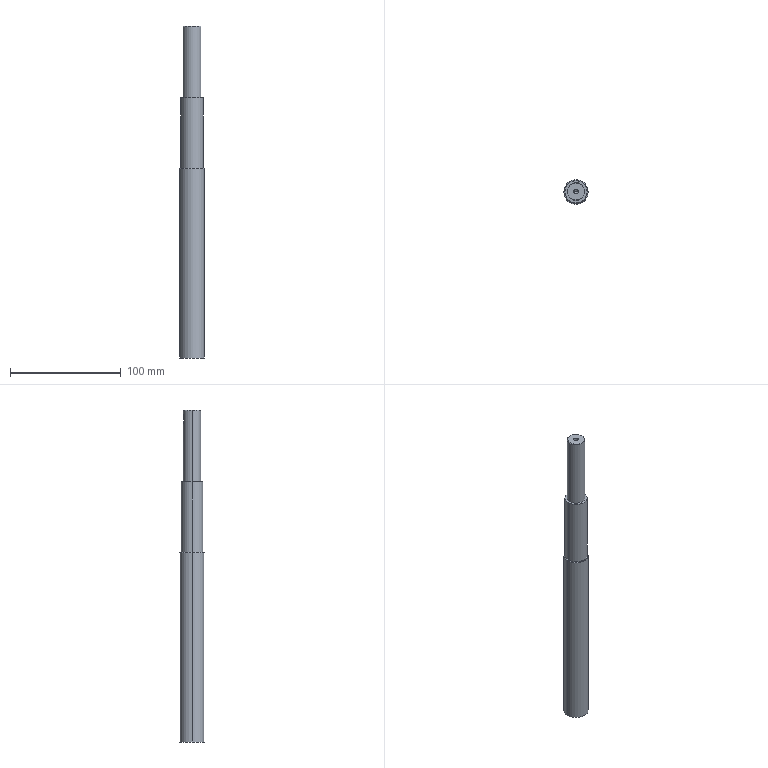Component | SolidWorks | UpperSideBeltRisingScrewXG-XG1-1 | 1 solid | 23 faces | box 22 x 22 x 300 mm | volume 97876 mm3 | cylinder 10 | plane 7 | cone 6 | commonest cylinder face diameters 4.2 x2 16 x2 20 x2 22 x2 5 x2
STEP:
#1=CARTESIAN_POINT('',(-13.812,18.504,15.591));
#2=VERTEX_POINT('',#1);
#3=CARTESIAN_POINT('',(-13.646,18.504,15.591));
#4=VERTEX_POINT('',#3);
#5=CARTESIAN_POINT('',(-13.729,18.504,15.591));
#6=DIRECTION('',(0.,-0.,1.));
#7=DIRECTION('',(1.,0.,0.));
#8=AXIS2_PLACEMENT_3D('',#5,#6,#7);
#9=CIRCLE('',#8,0.08268);
#10=EDGE_CURVE('',#2,#4,#9,.T.);
#11=ORIENTED_EDGE('',*,*,#10,.F.);
#12=CARTESIAN_POINT('',(-13.812,18.504,16.08));
#13=VERTEX_POINT('',#12);
#14=CARTESIAN_POINT('',(-13.812,18.504,16.08));
#15=DIRECTION('',(0.,-0.,1.));
#16=VECTOR('',#15,39.37);
#17=LINE('',#14,#16);
#18=EDGE_CURVE('',#2,#13,#17,.T.);
#19=ORIENTED_EDGE('',*,*,#18,.T.);
#20=CARTESIAN_POINT('',(-13.646,18.504,16.08));
#21=VERTEX_POINT('',#20);
#22=CARTESIAN_POINT('',(-13.729,18.504,16.08));
#23=DIRECTION('',(0.,-0.,1.));
#24=DIRECTION('',(1.,0.,0.));
#25=AXIS2_PLACEMENT_3D('',#22,#23,#24);
#26=CIRCLE('',#25,0.08268);
#27=EDGE_CURVE('',#13,#21,#26,.T.);
#28=ORIENTED_EDGE('',*,*,#27,.T.);
#29=CARTESIAN_POINT('',(-13.646,18.504,16.08));
#30=DIRECTION('',(0.,-0.,1.));
#31=VECTOR('',#30,39.37);
#32=LINE('',#29,#31);
#33=EDGE_CURVE('',#4,#21,#32,.T.);
#34=ORIENTED_EDGE('',*,*,#33,.F.);
#35=EDGE_LOOP('',(#11,#19,#28,#34));
#36=FACE_OUTER_BOUND('',#35,.T.);
#37=CARTESIAN_POINT('',(-13.729,18.504,16.08));
#38=DIRECTION('',(0.,-0.,1.));
#39=DIRECTION('',(1.,0.,0.));
#40=AXIS2_PLACEMENT_3D('',#37,#38,#39);
#41=CYLINDRICAL_SURFACE('',#40,0.08268);
#42=ADVANCED_FACE('',(#36),#41,.F.);
#43=CARTESIAN_POINT('',(-13.729,18.504,15.542));
#44=VERTEX_POINT('',#43);
#45=CARTESIAN_POINT('',(-13.646,18.504,15.591));
#46=DIRECTION('',(0.8572,-0.,0.515));
#47=VECTOR('',#46,39.37);
#48=LINE('',#45,#47);
#49=EDGE_CURVE('',#44,#4,#48,.T.);
#50=ORIENTED_EDGE('',*,*,#49,.F.);
#51=CARTESIAN_POINT('',(-13.812,18.504,15.591));
#52=DIRECTION('',(-0.8572,-0.,0.515));
#53=VECTOR('',#52,39.37);
#54=LINE('',#51,#53);
#55=EDGE_CURVE('',#44,#2,#54,.T.);
#56=ORIENTED_EDGE('',*,*,#55,.T.);
#57=ORIENTED_EDGE('',*,*,#10,.T.);
#58=EDGE_LOOP('',(#50,#56,#57));
#59=FACE_OUTER_BOUND('',#58,.T.);
#60=CARTESIAN_POINT('',(-13.729,18.504,15.591));
#61=DIRECTION('',(0.,-0.,1.));
#62=DIRECTION('',(1.,0.,0.));
#63=AXIS2_PLACEMENT_3D('',#60,#61,#62);
#64=CONICAL_SURFACE('',#63,0.08268,1.03);
#65=ADVANCED_FACE('',(#59),#64,.F.);
#66=CARTESIAN_POINT('',(-13.828,18.803,15.883));
#67=VERTEX_POINT('',#66);
#68=CARTESIAN_POINT('',(-13.828,18.803,15.646));
#69=VERTEX_POINT('',#68);
#70=CARTESIAN_POINT('',(-13.828,18.803,16.97));
#71=DIRECTION('',(-0.,0.,-1.));
#72=VECTOR('',#71,39.37);
#73=LINE('',#70,#72);
#74=EDGE_CURVE('',#67,#69,#73,.T.);
#75=ORIENTED_EDGE('',*,*,#74,.T.);
#76=CARTESIAN_POINT('',(-13.631,18.803,15.646));
#77=VERTEX_POINT('',#76);
#78=CARTESIAN_POINT('',(-13.828,18.803,15.646));
#79=CARTESIAN_POINT('',(-13.828,18.803,15.64));
#80=CARTESIAN_POINT('',(-13.827,18.803,15.634));
#81=CARTESIAN_POINT('',(-13.824,18.804,15.621));
#82=CARTESIAN_POINT('',(-13.822,18.805,15.615));
#83=CARTESIAN_POINT('',(-13.818,18.806,15.603));
#84=CARTESIAN_POINT('',(-13.814,18.807,15.597));
#85=CARTESIAN_POINT('',(-13.807,18.809,15.586));
#86=CARTESIAN_POINT('',(-13.803,18.81,15.581));
#87=CARTESIAN_POINT('',(-13.79,18.813,15.568));
#88=CARTESIAN_POINT('',(-13.779,18.815,15.561));
#89=CARTESIAN_POINT('',(-13.761,18.817,15.553));
#90=CARTESIAN_POINT('',(-13.755,18.818,15.551));
#91=CARTESIAN_POINT('',(-13.742,18.819,15.549));
#92=CARTESIAN_POINT('',(-13.736,18.819,15.548));
#93=CARTESIAN_POINT('',(-13.723,18.819,15.548));
#94=CARTESIAN_POINT('',(-13.716,18.819,15.549));
#95=CARTESIAN_POINT('',(-13.704,18.818,15.551));
#96=CARTESIAN_POINT('',(-13.697,18.817,15.553));
#97=CARTESIAN_POINT('',(-13.685,18.816,15.558));
#98=CARTESIAN_POINT('',(-13.68,18.815,15.561));
#99=CARTESIAN_POINT('',(-13.669,18.813,15.568));
#100=CARTESIAN_POINT('',(-13.664,18.812,15.572));
#101=CARTESIAN_POINT('',(-13.655,18.81,15.581));
#102=CARTESIAN_POINT('',(-13.651,18.809,15.586));
#103=CARTESIAN_POINT('',(-13.644,18.807,15.597));
#104=CARTESIAN_POINT('',(-13.641,18.806,15.603));
#105=CARTESIAN_POINT('',(-13.636,18.805,15.615));
#106=CARTESIAN_POINT('',(-13.634,18.804,15.621));
#107=CARTESIAN_POINT('',(-13.631,18.803,15.633));
#108=CARTESIAN_POINT('',(-13.631,18.803,15.64));
#109=CARTESIAN_POINT('',(-13.631,18.803,15.646));
#110=B_SPLINE_CURVE_WITH_KNOTS('',3,(#78,#79,#80,#81,#82,#83,#84,#85,#86,#87,#88,#89,#90,#91,#92,#93,#94,#95,#96,#97,#98,#99,#100,#101,#102,#103,#104,#105,#106,#107,#108,#109),.UNSPECIFIED.,.F.,.F.,(4,2,2,2,2,2,2,2,2,2,2,2,2,2,2,4),(0.,0.0004914,0.0009828,0.001474,0.001966,0.002949,0.00344,0.003931,0.004423,0.004914,0.005406,0.005897,0.006388,0.00688,0.007371,0.007863),.UNSPECIFIED.);
#111=EDGE_CURVE('',#69,#77,#110,.T.);
#112=ORIENTED_EDGE('',*,*,#111,.T.);
#113=CARTESIAN_POINT('',(-13.631,18.803,15.883));
#114=VERTEX_POINT('',#113);
#115=CARTESIAN_POINT('',(-13.631,18.803,16.97));
#116=DIRECTION('',(0.,-0.,1.));
#117=VECTOR('',#116,39.37);
#118=LINE('',#115,#117);
#119=EDGE_CURVE('',#77,#114,#118,.T.);
#120=ORIENTED_EDGE('',*,*,#119,.T.);
#121=CARTESIAN_POINT('',(-13.631,18.803,15.883));
#122=CARTESIAN_POINT('',(-13.631,18.803,15.889));
#123=CARTESIAN_POINT('',(-13.631,18.803,15.896));
#124=CARTESIAN_POINT('',(-13.634,18.804,15.908));
#125=CARTESIAN_POINT('',(-13.636,18.805,15.915));
#126=CARTESIAN_POINT('',(-13.641,18.806,15.926));
#127=CARTESIAN_POINT('',(-13.644,18.807,15.932));
#128=CARTESIAN_POINT('',(-13.651,18.809,15.943));
#129=CARTESIAN_POINT('',(-13.655,18.81,15.948));
#130=CARTESIAN_POINT('',(-13.669,18.813,15.961));
#131=CARTESIAN_POINT('',(-13.679,18.815,15.969));
#132=CARTESIAN_POINT('',(-13.697,18.817,15.976));
#133=CARTESIAN_POINT('',(-13.703,18.818,15.978));
#134=CARTESIAN_POINT('',(-13.716,18.819,15.98));
#135=CARTESIAN_POINT('',(-13.723,18.819,15.981));
#136=CARTESIAN_POINT('',(-13.735,18.819,15.981));
#137=CARTESIAN_POINT('',(-13.742,18.819,15.98));
#138=CARTESIAN_POINT('',(-13.755,18.818,15.978));
#139=CARTESIAN_POINT('',(-13.761,18.817,15.976));
#140=CARTESIAN_POINT('',(-13.773,18.816,15.971));
#141=CARTESIAN_POINT('',(-13.779,18.815,15.968));
#142=CARTESIAN_POINT('',(-13.789,18.813,15.961));
#143=CARTESIAN_POINT('',(-13.794,18.812,15.957));
#144=CARTESIAN_POINT('',(-13.803,18.81,15.948));
#145=CARTESIAN_POINT('',(-13.807,18.809,15.943));
#146=CARTESIAN_POINT('',(-13.814,18.807,15.932));
#147=CARTESIAN_POINT('',(-13.818,18.806,15.926));
#148=CARTESIAN_POINT('',(-13.822,18.805,15.915));
#149=CARTESIAN_POINT('',(-13.824,18.804,15.908));
#150=CARTESIAN_POINT('',(-13.827,18.803,15.896));
#151=CARTESIAN_POINT('',(-13.828,18.803,15.889));
#152=CARTESIAN_POINT('',(-13.828,18.803,15.883));
#153=B_SPLINE_CURVE_WITH_KNOTS('',3,(#121,#122,#123,#124,#125,#126,#127,#128,#129,#130,#131,#132,#133,#134,#135,#136,#137,#138,#139,#140,#141,#142,#143,#144,#145,#146,#147,#148,#149,#150,#151,#152),.UNSPECIFIED.,.F.,.F.,(4,2,2,2,2,2,2,2,2,2,2,2,2,2,2,4),(0.,0.0004914,0.0009828,0.001474,0.001966,0.002949,0.00344,0.003931,0.004423,0.004914,0.005406,0.005897,0.006388,0.00688,0.007371,0.007863),.UNSPECIFIED.);
#154=EDGE_CURVE('',#114,#67,#153,.T.);
#155=ORIENTED_EDGE('',*,*,#154,.T.);
#156=EDGE_LOOP('',(#75,#112,#120,#155));
#157=FACE_BOUND('',#156,.T.);
#158=CARTESIAN_POINT('',(-14.044,18.504,16.06));
#159=VERTEX_POINT('',#158);
#160=CARTESIAN_POINT('',(-13.414,18.504,16.06));
#161=VERTEX_POINT('',#160);
#162=CARTESIAN_POINT('',(-13.729,18.504,16.06));
#163=DIRECTION('',(-0.,0.,-1.));
#164=DIRECTION('',(1.,0.,0.));
#165=AXIS2_PLACEMENT_3D('',#162,#163,#164);
#166=CIRCLE('',#165,0.315);
#167=EDGE_CURVE('',#159,#161,#166,.T.);
#168=ORIENTED_EDGE('',*,*,#167,.T.);
#169=CARTESIAN_POINT('',(-13.414,18.504,13.52));
#170=VERTEX_POINT('',#169);
#171=CARTESIAN_POINT('',(-13.414,18.504,16.97));
#172=DIRECTION('',(-0.,0.,-1.));
#173=VECTOR('',#172,39.37);
#174=LINE('',#171,#173);
#175=EDGE_CURVE('',#161,#170,#174,.T.);
#176=ORIENTED_EDGE('',*,*,#175,.T.);
#177=CARTESIAN_POINT('',(-14.044,18.504,13.52));
#178=VERTEX_POINT('',#177);
#179=CARTESIAN_POINT('',(-13.729,18.504,13.52));
#180=DIRECTION('',(0.,-0.,1.));
#181=DIRECTION('',(1.,0.,0.));
#182=AXIS2_PLACEMENT_3D('',#179,#180,#181);
#183=CIRCLE('',#182,0.315);
#184=EDGE_CURVE('',#170,#178,#183,.T.);
#185=ORIENTED_EDGE('',*,*,#184,.T.);
#186=CARTESIAN_POINT('',(-14.044,18.504,16.97));
#187=DIRECTION('',(-0.,0.,-1.));
#188=VECTOR('',#187,39.37);
#189=LINE('',#186,#188);
#190=EDGE_CURVE('',#159,#178,#189,.T.);
#191=ORIENTED_EDGE('',*,*,#190,.F.);
#192=EDGE_LOOP('',(#168,#176,#185,#191));
#193=FACE_OUTER_BOUND('',#192,.T.);
#194=CARTESIAN_POINT('',(-13.729,18.504,16.97));
#195=DIRECTION('',(-0.,0.,-1.));
#196=DIRECTION('',(-1.,0.,0.));
#197=AXIS2_PLACEMENT_3D('',#194,#195,#196);
#198=CYLINDRICAL_SURFACE('',#197,0.315);
#199=ADVANCED_FACE('',(#157,#193),#198,.T.);
#200=CARTESIAN_POINT('',(-13.434,18.504,16.08));
#201=VERTEX_POINT('',#200);
#202=CARTESIAN_POINT('',(-14.024,18.504,16.08));
#203=VERTEX_POINT('',#202);
#204=CARTESIAN_POINT('',(-13.729,18.504,16.08));
#205=DIRECTION('',(0.,-0.,1.));
#206=DIRECTION('',(1.,0.,0.));
#207=AXIS2_PLACEMENT_3D('',#204,#205,#206);
#208=CIRCLE('',#207,0.2953);
#209=EDGE_CURVE('',#201,#203,#208,.T.);
#210=ORIENTED_EDGE('',*,*,#209,.F.);
#211=CARTESIAN_POINT('',(-13.434,18.504,16.08));
#212=DIRECTION('',(0.7071,0.,-0.7071));
#213=VECTOR('',#212,39.37);
#214=LINE('',#211,#213);
#215=EDGE_CURVE('',#201,#161,#214,.T.);
#216=ORIENTED_EDGE('',*,*,#215,.T.);
#217=ORIENTED_EDGE('',*,*,#167,.F.);
#218=CARTESIAN_POINT('',(-14.024,18.504,16.08));
#219=DIRECTION('',(-0.7071,0.,-0.7071));
#220=VECTOR('',#219,39.37);
#221=LINE('',#218,#220);
#222=EDGE_CURVE('',#203,#159,#221,.T.);
#223=ORIENTED_EDGE('',*,*,#222,.F.);
#224=EDGE_LOOP('',(#210,#216,#217,#223));
#225=FACE_OUTER_BOUND('',#224,.T.);
#226=CARTESIAN_POINT('',(-13.729,18.504,16.08));
#227=DIRECTION('',(-0.,0.,-1.));
#228=DIRECTION('',(-1.,0.,0.));
#229=AXIS2_PLACEMENT_3D('',#226,#227,#228);
#230=CONICAL_SURFACE('',#229,0.2953,0.7854);
#231=ADVANCED_FACE('',(#225),#230,.T.);
#232=CARTESIAN_POINT('',(-13.316,18.504,11.02));
#233=VERTEX_POINT('',#232);
#234=CARTESIAN_POINT('',(-14.143,18.504,11.02));
#235=VERTEX_POINT('',#234);
#236=CARTESIAN_POINT('',(-13.729,18.504,11.02));
#237=DIRECTION('',(0.,-0.,1.));
#238=DIRECTION('',(1.,0.,0.));
#239=AXIS2_PLACEMENT_3D('',#236,#237,#238);
#240=CIRCLE('',#239,0.4134);
#241=EDGE_CURVE('',#233,#235,#240,.T.);
#242=ORIENTED_EDGE('',*,*,#241,.F.);
#243=CARTESIAN_POINT('',(-13.296,18.504,11.001));
#244=VERTEX_POINT('',#243);
#245=CARTESIAN_POINT('',(-13.316,18.504,11.02));
#246=DIRECTION('',(0.7071,0.,-0.7071));
#247=VECTOR('',#246,39.37);
#248=LINE('',#245,#247);
#249=EDGE_CURVE('',#233,#244,#248,.T.);
#250=ORIENTED_EDGE('',*,*,#249,.T.);
#251=CARTESIAN_POINT('',(-14.162,18.504,11.001));
#252=VERTEX_POINT('',#251);
#253=CARTESIAN_POINT('',(-13.729,18.504,11.001));
#254=DIRECTION('',(-0.,0.,-1.));
#255=DIRECTION('',(1.,0.,0.));
#256=AXIS2_PLACEMENT_3D('',#253,#254,#255);
#257=CIRCLE('',#256,0.4331);
#258=EDGE_CURVE('',#252,#244,#257,.T.);
#259=ORIENTED_EDGE('',*,*,#258,.F.);
#260=CARTESIAN_POINT('',(-14.143,18.504,11.02));
#261=DIRECTION('',(-0.7071,0.,-0.7071));
#262=VECTOR('',#261,39.37);
#263=LINE('',#260,#262);
#264=EDGE_CURVE('',#235,#252,#263,.T.);
#265=ORIENTED_EDGE('',*,*,#264,.F.);
#266=EDGE_LOOP('',(#242,#250,#259,#265));
#267=FACE_OUTER_BOUND('',#266,.T.);
#268=CARTESIAN_POINT('',(-13.729,18.504,11.02));
#269=DIRECTION('',(-0.,0.,-1.));
#270=DIRECTION('',(-1.,0.,0.));
#271=AXIS2_PLACEMENT_3D('',#268,#269,#270);
#272=CONICAL_SURFACE('',#271,0.4134,0.7854);
#273=ADVANCED_FACE('',(#267),#272,.T.);
#274=CARTESIAN_POINT('',(-14.123,18.504,11.02));
#275=VERTEX_POINT('',#274);
#276=CARTESIAN_POINT('',(-13.335,18.504,11.02));
#277=VERTEX_POINT('',#276);
#278=CARTESIAN_POINT('',(-13.729,18.504,11.02));
#279=DIRECTION('',(-0.,0.,-1.));
#280=DIRECTION('',(-1.,0.,0.));
#281=AXIS2_PLACEMENT_3D('',#278,#279,#280);
#282=CIRCLE('',#281,0.3937);
#283=EDGE_CURVE('',#275,#277,#282,.T.);
#284=ORIENTED_EDGE('',*,*,#283,.F.);
#285=CARTESIAN_POINT('',(-14.123,18.504,13.52));
#286=VERTEX_POINT('',#285);
#287=CARTESIAN_POINT('',(-14.123,18.504,15.41));
#288=DIRECTION('',(0.,-0.,1.));
#289=VECTOR('',#288,39.37);
#290=LINE('',#287,#289);
#291=EDGE_CURVE('',#275,#286,#290,.T.);
#292=ORIENTED_EDGE('',*,*,#291,.T.);
#293=CARTESIAN_POINT('',(-13.335,18.504,13.52));
#294=VERTEX_POINT('',#293);
#295=CARTESIAN_POINT('',(-13.729,18.504,13.52));
#296=DIRECTION('',(0.,-0.,1.));
#297=DIRECTION('',(1.,0.,0.));
#298=AXIS2_PLACEMENT_3D('',#295,#296,#297);
#299=CIRCLE('',#298,0.3937);
#300=EDGE_CURVE('',#294,#286,#299,.T.);
#301=ORIENTED_EDGE('',*,*,#300,.F.);
#302=CARTESIAN_POINT('',(-13.335,18.504,15.41));
#303=DIRECTION('',(0.,-0.,1.));
#304=VECTOR('',#303,39.37);
#305=LINE('',#302,#304);
#306=EDGE_CURVE('',#277,#294,#305,.T.);
#307=ORIENTED_EDGE('',*,*,#306,.F.);
#308=EDGE_LOOP('',(#284,#292,#301,#307));
#309=FACE_OUTER_BOUND('',#308,.T.);
#310=CARTESIAN_POINT('',(-13.729,18.504,15.41));
#311=DIRECTION('',(0.,-0.,1.));
#312=DIRECTION('',(1.,0.,0.));
#313=AXIS2_PLACEMENT_3D('',#310,#311,#312);
#314=CYLINDRICAL_SURFACE('',#313,0.3937);
#315=ADVANCED_FACE('',(#309),#314,.T.);
#316=ORIENTED_EDGE('',*,*,#258,.T.);
#317=CARTESIAN_POINT('',(-13.296,18.504,4.269));
#318=VERTEX_POINT('',#317);
#319=CARTESIAN_POINT('',(-13.296,18.504,16.08));
#320=DIRECTION('',(-0.,0.,-1.));
#321=VECTOR('',#320,39.37);
#322=LINE('',#319,#321);
#323=EDGE_CURVE('',#244,#318,#322,.T.);
#324=ORIENTED_EDGE('',*,*,#323,.T.);
#325=CARTESIAN_POINT('',(-14.162,18.504,4.269));
#326=VERTEX_POINT('',#325);
#327=CARTESIAN_POINT('',(-13.729,18.504,4.269));
#328=DIRECTION('',(-0.,0.,-1.));
#329=DIRECTION('',(-1.,0.,0.));
#330=AXIS2_PLACEMENT_3D('',#327,#328,#329);
#331=CIRCLE('',#330,0.4331);
#332=EDGE_CURVE('',#326,#318,#331,.T.);
#333=ORIENTED_EDGE('',*,*,#332,.F.);
#334=CARTESIAN_POINT('',(-14.162,18.504,16.08));
#335=DIRECTION('',(-0.,0.,-1.));
#336=VECTOR('',#335,39.37);
#337=LINE('',#334,#336);
#338=EDGE_CURVE('',#252,#326,#337,.T.);
#339=ORIENTED_EDGE('',*,*,#338,.F.);
#340=EDGE_LOOP('',(#316,#324,#333,#339));
#341=FACE_OUTER_BOUND('',#340,.T.);
#342=CARTESIAN_POINT('',(-13.729,18.504,16.08));
#343=DIRECTION('',(-0.,0.,-1.));
#344=DIRECTION('',(-1.,0.,0.));
#345=AXIS2_PLACEMENT_3D('',#342,#343,#344);
#346=CYLINDRICAL_SURFACE('',#345,0.4331);
#347=ADVANCED_FACE('',(#341),#346,.T.);
#348=ORIENTED_EDGE('',*,*,#323,.F.);
#349=CARTESIAN_POINT('',(-13.729,18.504,11.001));
#350=DIRECTION('',(-0.,0.,-1.));
#351=DIRECTION('',(1.,0.,0.));
#352=AXIS2_PLACEMENT_3D('',#349,#350,#351);
#353=CIRCLE('',#352,0.4331);
#354=EDGE_CURVE('',#244,#252,#353,.T.);
#355=ORIENTED_EDGE('',*,*,#354,.T.);
#356=ORIENTED_EDGE('',*,*,#338,.T.);
#357=CARTESIAN_POINT('',(-13.729,18.504,4.269));
#358=DIRECTION('',(-0.,0.,-1.));
#359=DIRECTION('',(-1.,0.,0.));
#360=AXIS2_PLACEMENT_3D('',#357,#358,#359);
#361=CIRCLE('',#360,0.4331);
#362=EDGE_CURVE('',#318,#326,#361,.T.);
#363=ORIENTED_EDGE('',*,*,#362,.F.);
#364=EDGE_LOOP('',(#348,#355,#356,#363));
#365=FACE_OUTER_BOUND('',#364,.T.);
#366=CARTESIAN_POINT('',(-13.729,18.504,16.08));
#367=DIRECTION('',(-0.,0.,-1.));
#368=DIRECTION('',(-1.,0.,0.));
#369=AXIS2_PLACEMENT_3D('',#366,#367,#368);
#370=CYLINDRICAL_SURFACE('',#369,0.4331);
#371=ADVANCED_FACE('',(#365),#370,.T.);
#372=ORIENTED_EDGE('',*,*,#291,.F.);
#373=CARTESIAN_POINT('',(-13.729,18.504,11.02));
#374=DIRECTION('',(-0.,0.,-1.));
#375=DIRECTION('',(-1.,0.,0.));
#376=AXIS2_PLACEMENT_3D('',#373,#374,#375);
#377=CIRCLE('',#376,0.3937);
#378=EDGE_CURVE('',#277,#275,#377,.T.);
#379=ORIENTED_EDGE('',*,*,#378,.F.);
#380=ORIENTED_EDGE('',*,*,#306,.T.);
#381=CARTESIAN_POINT('',(-13.729,18.504,13.52));
#382=DIRECTION('',(0.,-0.,1.));
#383=DIRECTION('',(1.,0.,0.));
#384=AXIS2_PLACEMENT_3D('',#381,#382,#383);
#385=CIRCLE('',#384,0.3937);
#386=EDGE_CURVE('',#286,#294,#385,.T.);
#387=ORIENTED_EDGE('',*,*,#386,.F.);
#388=EDGE_LOOP('',(#372,#379,#380,#387));
#389=FACE_OUTER_BOUND('',#388,.T.);
#390=CARTESIAN_POINT('',(-13.729,18.504,15.41));
#391=DIRECTION('',(0.,-0.,1.));
#392=DIRECTION('',(1.,0.,0.));
#393=AXIS2_PLACEMENT_3D('',#390,#391,#392);
#394=CYLINDRICAL_SURFACE('',#393,0.3937);
#395=ADVANCED_FACE('',(#389),#394,.T.);
#396=CARTESIAN_POINT('',(-13.729,18.504,11.02));
#397=DIRECTION('',(0.,-0.,1.));
#398=DIRECTION('',(1.,0.,0.));
#399=AXIS2_PLACEMENT_3D('',#396,#397,#398);
#400=CIRCLE('',#399,0.4134);
#401=EDGE_CURVE('',#235,#233,#400,.T.);
#402=ORIENTED_EDGE('',*,*,#401,.T.);
#403=ORIENTED_EDGE('',*,*,#241,.T.);
#404=EDGE_LOOP('',(#402,#403));
#405=FACE_OUTER_BOUND('',#404,.T.);
#406=ORIENTED_EDGE('',*,*,#378,.T.);
#407=ORIENTED_EDGE('',*,*,#283,.T.);
#408=EDGE_LOOP('',(#406,#407));
#409=FACE_BOUND('',#408,.T.);
#410=CARTESIAN_POINT('',(-12.524,18.504,11.02));
#411=DIRECTION('',(0.,-0.,1.));
#412=DIRECTION('',(1.,0.,-0.));
#413=AXIS2_PLACEMENT_3D('',#410,#411,#412);
#414=PLANE('',#413);
#415=ADVANCED_FACE('',(#405,#409),#414,.T.);
#416=ORIENTED_EDGE('',*,*,#249,.F.);
#417=ORIENTED_EDGE('',*,*,#401,.F.);
#418=ORIENTED_EDGE('',*,*,#264,.T.);
#419=ORIENTED_EDGE('',*,*,#354,.F.);
#420=EDGE_LOOP('',(#416,#417,#418,#419));
#421=FACE_OUTER_BOUND('',#420,.T.);
#422=CARTESIAN_POINT('',(-13.729,18.504,11.02));
#423=DIRECTION('',(-0.,0.,-1.));
#424=DIRECTION('',(-1.,0.,0.));
#425=AXIS2_PLACEMENT_3D('',#422,#423,#424);
#426=CONICAL_SURFACE('',#425,0.4134,0.7854);
#427=ADVANCED_FACE('',(#421),#426,.T.);
#428=CARTESIAN_POINT('',(-13.729,18.504,13.52));
#429=DIRECTION('',(0.,-0.,1.));
#430=DIRECTION('',(1.,0.,0.));
#431=AXIS2_PLACEMENT_3D('',#428,#429,#430);
#432=CIRCLE('',#431,0.315);
#433=EDGE_CURVE('',#178,#170,#432,.T.);
#434=ORIENTED_EDGE('',*,*,#433,.F.);
#435=ORIENTED_EDGE('',*,*,#184,.F.);
#436=EDGE_LOOP('',(#434,#435));
#437=FACE_BOUND('',#436,.T.);
#438=ORIENTED_EDGE('',*,*,#300,.T.);
#439=ORIENTED_EDGE('',*,*,#386,.T.);
#440=EDGE_LOOP('',(#438,#439));
#441=FACE_OUTER_BOUND('',#440,.T.);
#442=CARTESIAN_POINT('',(-13.729,18.504,13.52));
#443=DIRECTION('',(0.,-0.,1.));
#444=DIRECTION('',(1.,0.,-0.));
#445=AXIS2_PLACEMENT_3D('',#442,#443,#444);
#446=PLANE('',#445);
#447=ADVANCED_FACE('',(#437,#441),#446,.T.);
#448=CARTESIAN_POINT('',(-13.729,18.504,16.08));
#449=DIRECTION('',(0.,-0.,1.));
#450=DIRECTION('',(1.,0.,0.));
#451=AXIS2_PLACEMENT_3D('',#448,#449,#450);
#452=CIRCLE('',#451,0.08268);
#453=EDGE_CURVE('',#21,#13,#452,.T.);
#454=ORIENTED_EDGE('',*,*,#453,.F.);
#455=ORIENTED_EDGE('',*,*,#27,.F.);
#456=EDGE_LOOP('',(#454,#455));
#457=FACE_BOUND('',#456,.T.);
#458=CARTESIAN_POINT('',(-13.729,18.504,16.08));
#459=DIRECTION('',(0.,-0.,1.));
#460=DIRECTION('',(1.,0.,0.));
#461=AXIS2_PLACEMENT_3D('',#458,#459,#460);
#462=CIRCLE('',#461,0.2953);
#463=EDGE_CURVE('',#203,#201,#462,.T.);
#464=ORIENTED_EDGE('',*,*,#463,.T.);
#465=ORIENTED_EDGE('',*,*,#209,.T.);
#466=EDGE_LOOP('',(#464,#465));
#467=FACE_OUTER_BOUND('',#466,.T.);
#468=CARTESIAN_POINT('',(-13.729,18.504,16.08));
#469=DIRECTION('',(0.,-0.,1.));
#470=DIRECTION('',(1.,0.,-0.));
#471=AXIS2_PLACEMENT_3D('',#468,#469,#470);
#472=PLANE('',#471);
#473=ADVANCED_FACE('',(#457,#467),#472,.T.);
#474=ORIENTED_EDGE('',*,*,#215,.F.);
#475=ORIENTED_EDGE('',*,*,#463,.F.);
#476=ORIENTED_EDGE('',*,*,#222,.T.);
#477=CARTESIAN_POINT('',(-13.729,18.504,16.06));
#478=DIRECTION('',(-0.,0.,-1.));
#479=DIRECTION('',(1.,0.,0.));
#480=AXIS2_PLACEMENT_3D('',#477,#478,#479);
#481=CIRCLE('',#480,0.315);
#482=EDGE_CURVE('',#161,#159,#481,.T.);
#483=ORIENTED_EDGE('',*,*,#482,.F.);
#484=EDGE_LOOP('',(#474,#475,#476,#483));
#485=FACE_OUTER_BOUND('',#484,.T.);
#486=CARTESIAN_POINT('',(-13.729,18.504,16.08));
#487=DIRECTION('',(-0.,0.,-1.));
#488=DIRECTION('',(-1.,0.,0.));
#489=AXIS2_PLACEMENT_3D('',#486,#487,#488);
#490=CONICAL_SURFACE('',#489,0.2953,0.7854);
#491=ADVANCED_FACE('',(#485),#490,.T.);
#492=ORIENTED_EDGE('',*,*,#175,.F.);
#493=ORIENTED_EDGE('',*,*,#482,.T.);
#494=ORIENTED_EDGE('',*,*,#190,.T.);
#495=ORIENTED_EDGE('',*,*,#433,.T.);
#496=EDGE_LOOP('',(#492,#493,#494,#495));
#497=FACE_OUTER_BOUND('',#496,.T.);
#498=CARTESIAN_POINT('',(-13.729,18.504,16.97));
#499=DIRECTION('',(-0.,0.,-1.));
#500=DIRECTION('',(-1.,0.,0.));
#501=AXIS2_PLACEMENT_3D('',#498,#499,#500);
#502=CYLINDRICAL_SURFACE('',#501,0.315);
#503=ADVANCED_FACE('',(#497),#502,.T.);
#504=CARTESIAN_POINT('',(-13.631,18.701,15.883));
#505=VERTEX_POINT('',#504);
#506=CARTESIAN_POINT('',(-13.631,18.701,15.883));
#507=DIRECTION('',(-0.,1.,0.));
#508=VECTOR('',#507,39.37);
#509=LINE('',#506,#508);
#510=EDGE_CURVE('',#505,#114,#509,.T.);
#511=ORIENTED_EDGE('',*,*,#510,.F.);
#512=CARTESIAN_POINT('',(-13.828,18.701,15.883));
#513=VERTEX_POINT('',#512);
#514=CARTESIAN_POINT('',(-13.729,18.701,15.883));
#515=DIRECTION('',(-0.,1.,0.));
#516=DIRECTION('',(-1.,0.,0.));
#517=AXIS2_PLACEMENT_3D('',#514,#515,#516);
#518=CIRCLE('',#517,0.09843);
#519=EDGE_CURVE('',#513,#505,#518,.T.);
#520=ORIENTED_EDGE('',*,*,#519,.F.);
#521=CARTESIAN_POINT('',(-13.828,18.701,15.883));
#522=DIRECTION('',(-0.,1.,0.));
#523=VECTOR('',#522,39.37);
#524=LINE('',#521,#523);
#525=EDGE_CURVE('',#513,#67,#524,.T.);
#526=ORIENTED_EDGE('',*,*,#525,.T.);
#527=ORIENTED_EDGE('',*,*,#154,.F.);
#528=EDGE_LOOP('',(#511,#520,#526,#527));
#529=FACE_OUTER_BOUND('',#528,.T.);
#530=CARTESIAN_POINT('',(-13.729,18.701,15.883));
#531=DIRECTION('',(-0.,1.,0.));
#532=DIRECTION('',(-1.,0.,0.));
#533=AXIS2_PLACEMENT_3D('',#530,#531,#532);
#534=CYLINDRICAL_SURFACE('',#533,0.09843);
#535=ADVANCED_FACE('',(#529),#534,.F.);
#536=ORIENTED_EDGE('',*,*,#525,.F.);
#537=CARTESIAN_POINT('',(-13.828,18.701,15.646));
#538=VERTEX_POINT('',#537);
#539=CARTESIAN_POINT('',(-13.828,18.701,15.883));
#540=DIRECTION('',(0.,-0.,1.));
#541=VECTOR('',#540,39.37);
#542=LINE('',#539,#541);
#543=EDGE_CURVE('',#538,#513,#542,.T.);
#544=ORIENTED_EDGE('',*,*,#543,.F.);
#545=CARTESIAN_POINT('',(-13.828,18.701,15.646));
#546=DIRECTION('',(-0.,1.,0.));
#547=VECTOR('',#546,39.37);
#548=LINE('',#545,#547);
#549=EDGE_CURVE('',#538,#69,#548,.T.);
#550=ORIENTED_EDGE('',*,*,#549,.T.);
#551=ORIENTED_EDGE('',*,*,#74,.F.);
#552=EDGE_LOOP('',(#536,#544,#550,#551));
#553=FACE_OUTER_BOUND('',#552,.T.);
#554=CARTESIAN_POINT('',(-13.828,18.701,15.883));
#555=DIRECTION('',(-1.,-0.,0.));
#556=DIRECTION('',(0.,-0.,1.));
#557=AXIS2_PLACEMENT_3D('',#554,#555,#556);
#558=PLANE('',#557);
#559=ADVANCED_FACE('',(#553),#558,.F.);
#560=ORIENTED_EDGE('',*,*,#549,.F.);
#561=CARTESIAN_POINT('',(-13.631,18.701,15.646));
#562=VERTEX_POINT('',#561);
#563=CARTESIAN_POINT('',(-13.729,18.701,15.646));
#564=DIRECTION('',(-0.,1.,0.));
#565=DIRECTION('',(-1.,0.,0.));
#566=AXIS2_PLACEMENT_3D('',#563,#564,#565);
#567=CIRCLE('',#566,0.09843);
#568=EDGE_CURVE('',#562,#538,#567,.T.);
#569=ORIENTED_EDGE('',*,*,#568,.F.);
#570=CARTESIAN_POINT('',(-13.631,18.701,15.646));
#571=DIRECTION('',(-0.,1.,0.));
#572=VECTOR('',#571,39.37);
#573=LINE('',#570,#572);
#574=EDGE_CURVE('',#562,#77,#573,.T.);
#575=ORIENTED_EDGE('',*,*,#574,.T.);
#576=ORIENTED_EDGE('',*,*,#111,.F.);
#577=EDGE_LOOP('',(#560,#569,#575,#576));
#578=FACE_OUTER_BOUND('',#577,.T.);
#579=CARTESIAN_POINT('',(-13.729,18.701,15.646));
#580=DIRECTION('',(-0.,1.,0.));
#581=DIRECTION('',(-1.,0.,0.));
#582=AXIS2_PLACEMENT_3D('',#579,#580,#581);
#583=CYLINDRICAL_SURFACE('',#582,0.09843);
#584=ADVANCED_FACE('',(#578),#583,.F.);
#585=ORIENTED_EDGE('',*,*,#574,.F.);
#586=CARTESIAN_POINT('',(-13.631,18.701,15.883));
#587=DIRECTION('',(-0.,0.,-1.));
#588=VECTOR('',#587,39.37);
#589=LINE('',#586,#588);
#590=EDGE_CURVE('',#505,#562,#589,.T.);
#591=ORIENTED_EDGE('',*,*,#590,.F.);
#592=ORIENTED_EDGE('',*,*,#510,.T.);
#593=ORIENTED_EDGE('',*,*,#119,.F.);
#594=EDGE_LOOP('',(#585,#591,#592,#593));
#595=FACE_OUTER_BOUND('',#594,.T.);
#596=CARTESIAN_POINT('',(-13.631,18.701,15.883));
#597=DIRECTION('',(1.,0.,-0.));
#598=DIRECTION('',(-0.,0.,-1.));
#599=AXIS2_PLACEMENT_3D('',#596,#597,#598);
#600=PLANE('',#599);
#601=ADVANCED_FACE('',(#595),#600,.F.);
#602=ORIENTED_EDGE('',*,*,#519,.T.);
#603=ORIENTED_EDGE('',*,*,#590,.T.);
#604=ORIENTED_EDGE('',*,*,#568,.T.);
#605=ORIENTED_EDGE('',*,*,#543,.T.);
#606=EDGE_LOOP('',(#602,#603,#604,#605));
#607=FACE_OUTER_BOUND('',#606,.T.);
#608=CARTESIAN_POINT('',(-13.729,18.701,15.883));
#609=DIRECTION('',(-0.,1.,0.));
#610=DIRECTION('',(-1.,-0.,0.));
#611=AXIS2_PLACEMENT_3D('',#608,#609,#610);
#612=PLANE('',#611);
#613=ADVANCED_FACE('',(#607),#612,.T.);
#614=ORIENTED_EDGE('',*,*,#55,.F.);
#615=ORIENTED_EDGE('',*,*,#49,.T.);
#616=CARTESIAN_POINT('',(-13.729,18.504,15.591));
#617=DIRECTION('',(0.,-0.,1.));
#618=DIRECTION('',(1.,0.,0.));
#619=AXIS2_PLACEMENT_3D('',#616,#617,#618);
#620=CIRCLE('',#619,0.08268);
#621=EDGE_CURVE('',#4,#2,#620,.T.);
#622=ORIENTED_EDGE('',*,*,#621,.T.);
#623=EDGE_LOOP('',(#614,#615,#622));
#624=FACE_OUTER_BOUND('',#623,.T.);
#625=CARTESIAN_POINT('',(-13.729,18.504,15.591));
#626=DIRECTION('',(0.,-0.,1.));
#627=DIRECTION('',(1.,0.,0.));
#628=AXIS2_PLACEMENT_3D('',#625,#626,#627);
#629=CONICAL_SURFACE('',#628,0.08268,1.03);
#630=ADVANCED_FACE('',(#624),#629,.F.);
#631=ORIENTED_EDGE('',*,*,#18,.F.);
#632=ORIENTED_EDGE('',*,*,#621,.F.);
#633=ORIENTED_EDGE('',*,*,#33,.T.);
#634=ORIENTED_EDGE('',*,*,#453,.T.);
#635=EDGE_LOOP('',(#631,#632,#633,#634));
#636=FACE_OUTER_BOUND('',#635,.T.);
#637=CARTESIAN_POINT('',(-13.729,18.504,16.08));
#638=DIRECTION('',(0.,-0.,1.));
#639=DIRECTION('',(1.,0.,0.));
#640=AXIS2_PLACEMENT_3D('',#637,#638,#639);
#641=CYLINDRICAL_SURFACE('',#640,0.08268);
#642=ADVANCED_FACE('',(#636),#641,.F.);
#643=ORIENTED_EDGE('',*,*,#332,.T.);
#644=ORIENTED_EDGE('',*,*,#362,.T.);
#645=EDGE_LOOP('',(#643,#644));
#646=FACE_OUTER_BOUND('',#645,.T.);
#647=CARTESIAN_POINT('',(-13.729,18.504,4.269));
#648=DIRECTION('',(-0.,0.,-1.));
#649=DIRECTION('',(-1.,-0.,0.));
#650=AXIS2_PLACEMENT_3D('',#647,#648,#649);
#651=PLANE('',#650);
#652=ADVANCED_FACE('',(#646),#651,.T.);
#653=CLOSED_SHELL('',(#42,#65,#199,#231,#273,#315,#347,#371,#395,#415,#427,#447,#473,#491,#503,#535,#559,#584,#601,#613,#630,#642,#652));
#654=MANIFOLD_SOLID_BREP('',#653);
#655=CARTESIAN_POINT('',(0.,0.,0.));
#656=DIRECTION('',(0.,0.,1.));
#657=DIRECTION('',(1.,0.,0.));
#658=AXIS2_PLACEMENT_3D('',#655,#656,#657);
#659=(LENGTH_UNIT()NAMED_UNIT(*)SI_UNIT($,.METRE.));
#660=LENGTH_MEASURE_WITH_UNIT(LENGTH_MEASURE(0.0254),#659);
#661=DIMENSIONAL_EXPONENTS(1.,0.,0.,0.,0.,0.,0.);
#662=(CONVERSION_BASED_UNIT('',#660)LENGTH_UNIT()NAMED_UNIT(#661));
#663=UNCERTAINTY_MEASURE_WITH_UNIT(LENGTH_MEASURE(0.00001),#662,'','');
#664=(NAMED_UNIT(*)PLANE_ANGLE_UNIT()SI_UNIT($,.RADIAN.));
#665=(NAMED_UNIT(*)SI_UNIT($,.STERADIAN.)SOLID_ANGLE_UNIT());
#666=(GEOMETRIC_REPRESENTATION_CONTEXT(3)GLOBAL_UNCERTAINTY_ASSIGNED_CONTEXT((#663))GLOBAL_UNIT_ASSIGNED_CONTEXT((#662,#664,#665))REPRESENTATION_CONTEXT('',''));
#667=ADVANCED_BREP_SHAPE_REPRESENTATION('',(#654,#658),#666);
#668=COLOUR_RGB('',0.7922,0.8196,0.9333);
#669=FILL_AREA_STYLE_COLOUR('',#668);
#670=FILL_AREA_STYLE('',(#669));
#671=SURFACE_STYLE_FILL_AREA(#670);
#672=SURFACE_SIDE_STYLE('',(#671));
#673=SURFACE_STYLE_USAGE(.BOTH.,#672);
#674=PRESENTATION_STYLE_ASSIGNMENT((#673));
#675=STYLED_ITEM('',(#674),#654);
#676=(LENGTH_UNIT()NAMED_UNIT(*)SI_UNIT($,.METRE.));
#677=LENGTH_MEASURE_WITH_UNIT(LENGTH_MEASURE(0.0254),#676);
#678=DIMENSIONAL_EXPONENTS(1.,0.,0.,0.,0.,0.,0.);
#679=(CONVERSION_BASED_UNIT('',#677)LENGTH_UNIT()NAMED_UNIT(#678));
#680=UNCERTAINTY_MEASURE_WITH_UNIT(LENGTH_MEASURE(0.00001),#679,'','');
#681=(NAMED_UNIT(*)PLANE_ANGLE_UNIT()SI_UNIT($,.RADIAN.));
#682=(NAMED_UNIT(*)SI_UNIT($,.STERADIAN.)SOLID_ANGLE_UNIT());
#683=(GEOMETRIC_REPRESENTATION_CONTEXT(3)GLOBAL_UNCERTAINTY_ASSIGNED_CONTEXT((#680))GLOBAL_UNIT_ASSIGNED_CONTEXT((#679,#681,#682))REPRESENTATION_CONTEXT('',''));
#684=MECHANICAL_DESIGN_GEOMETRIC_PRESENTATION_REPRESENTATION('',(#675),#683);
#685=PRESENTATION_LAYER_ASSIGNMENT('','',(#675));